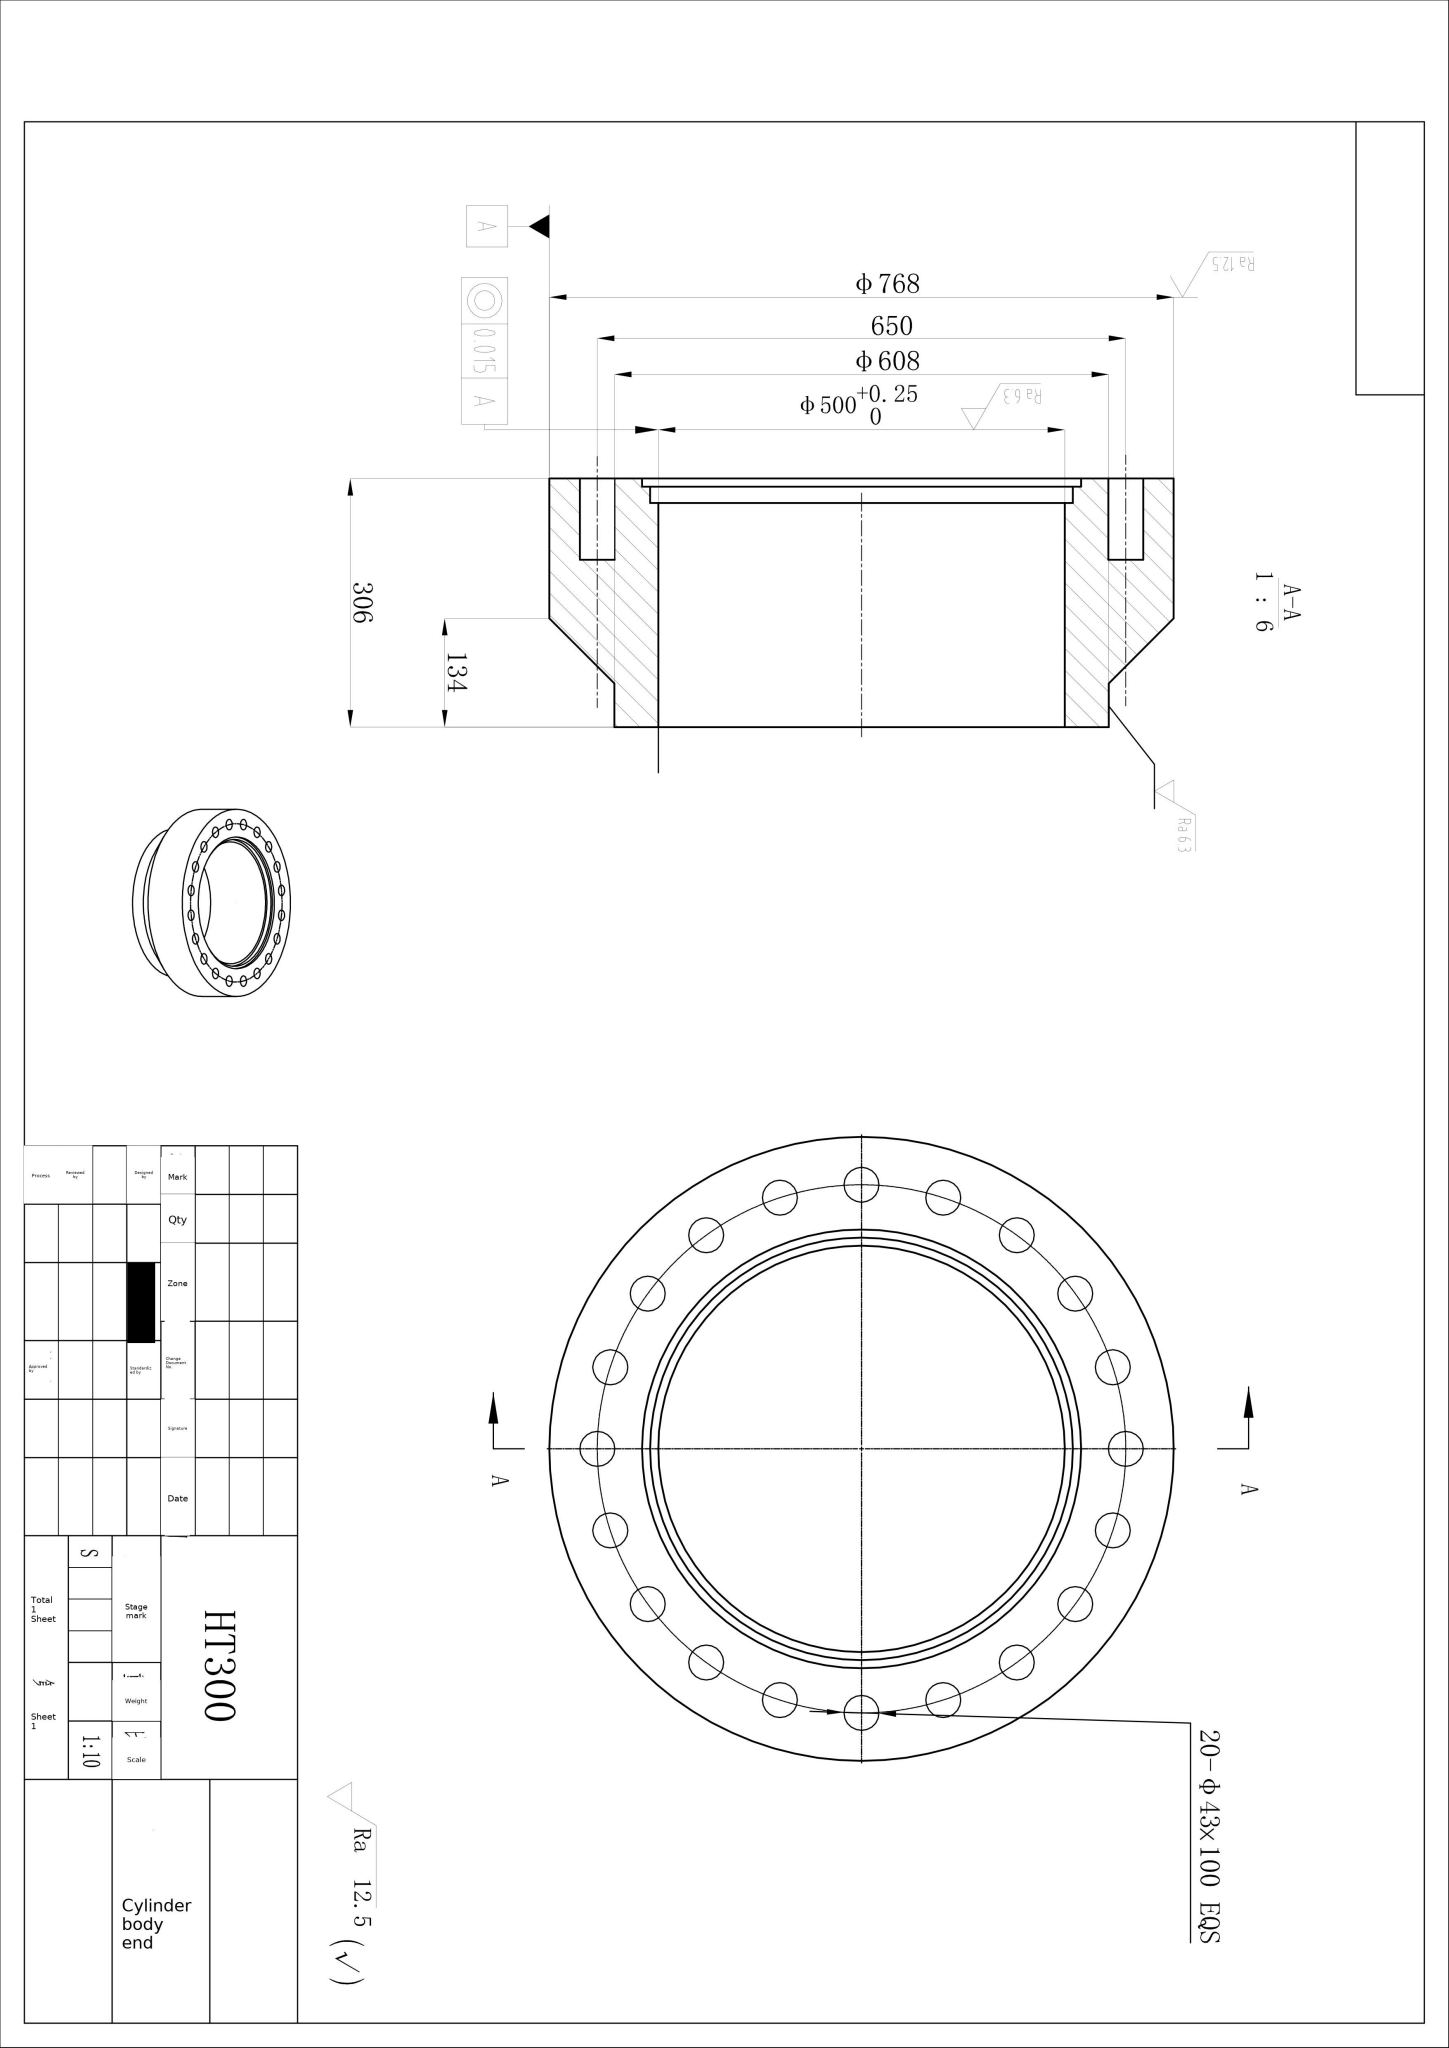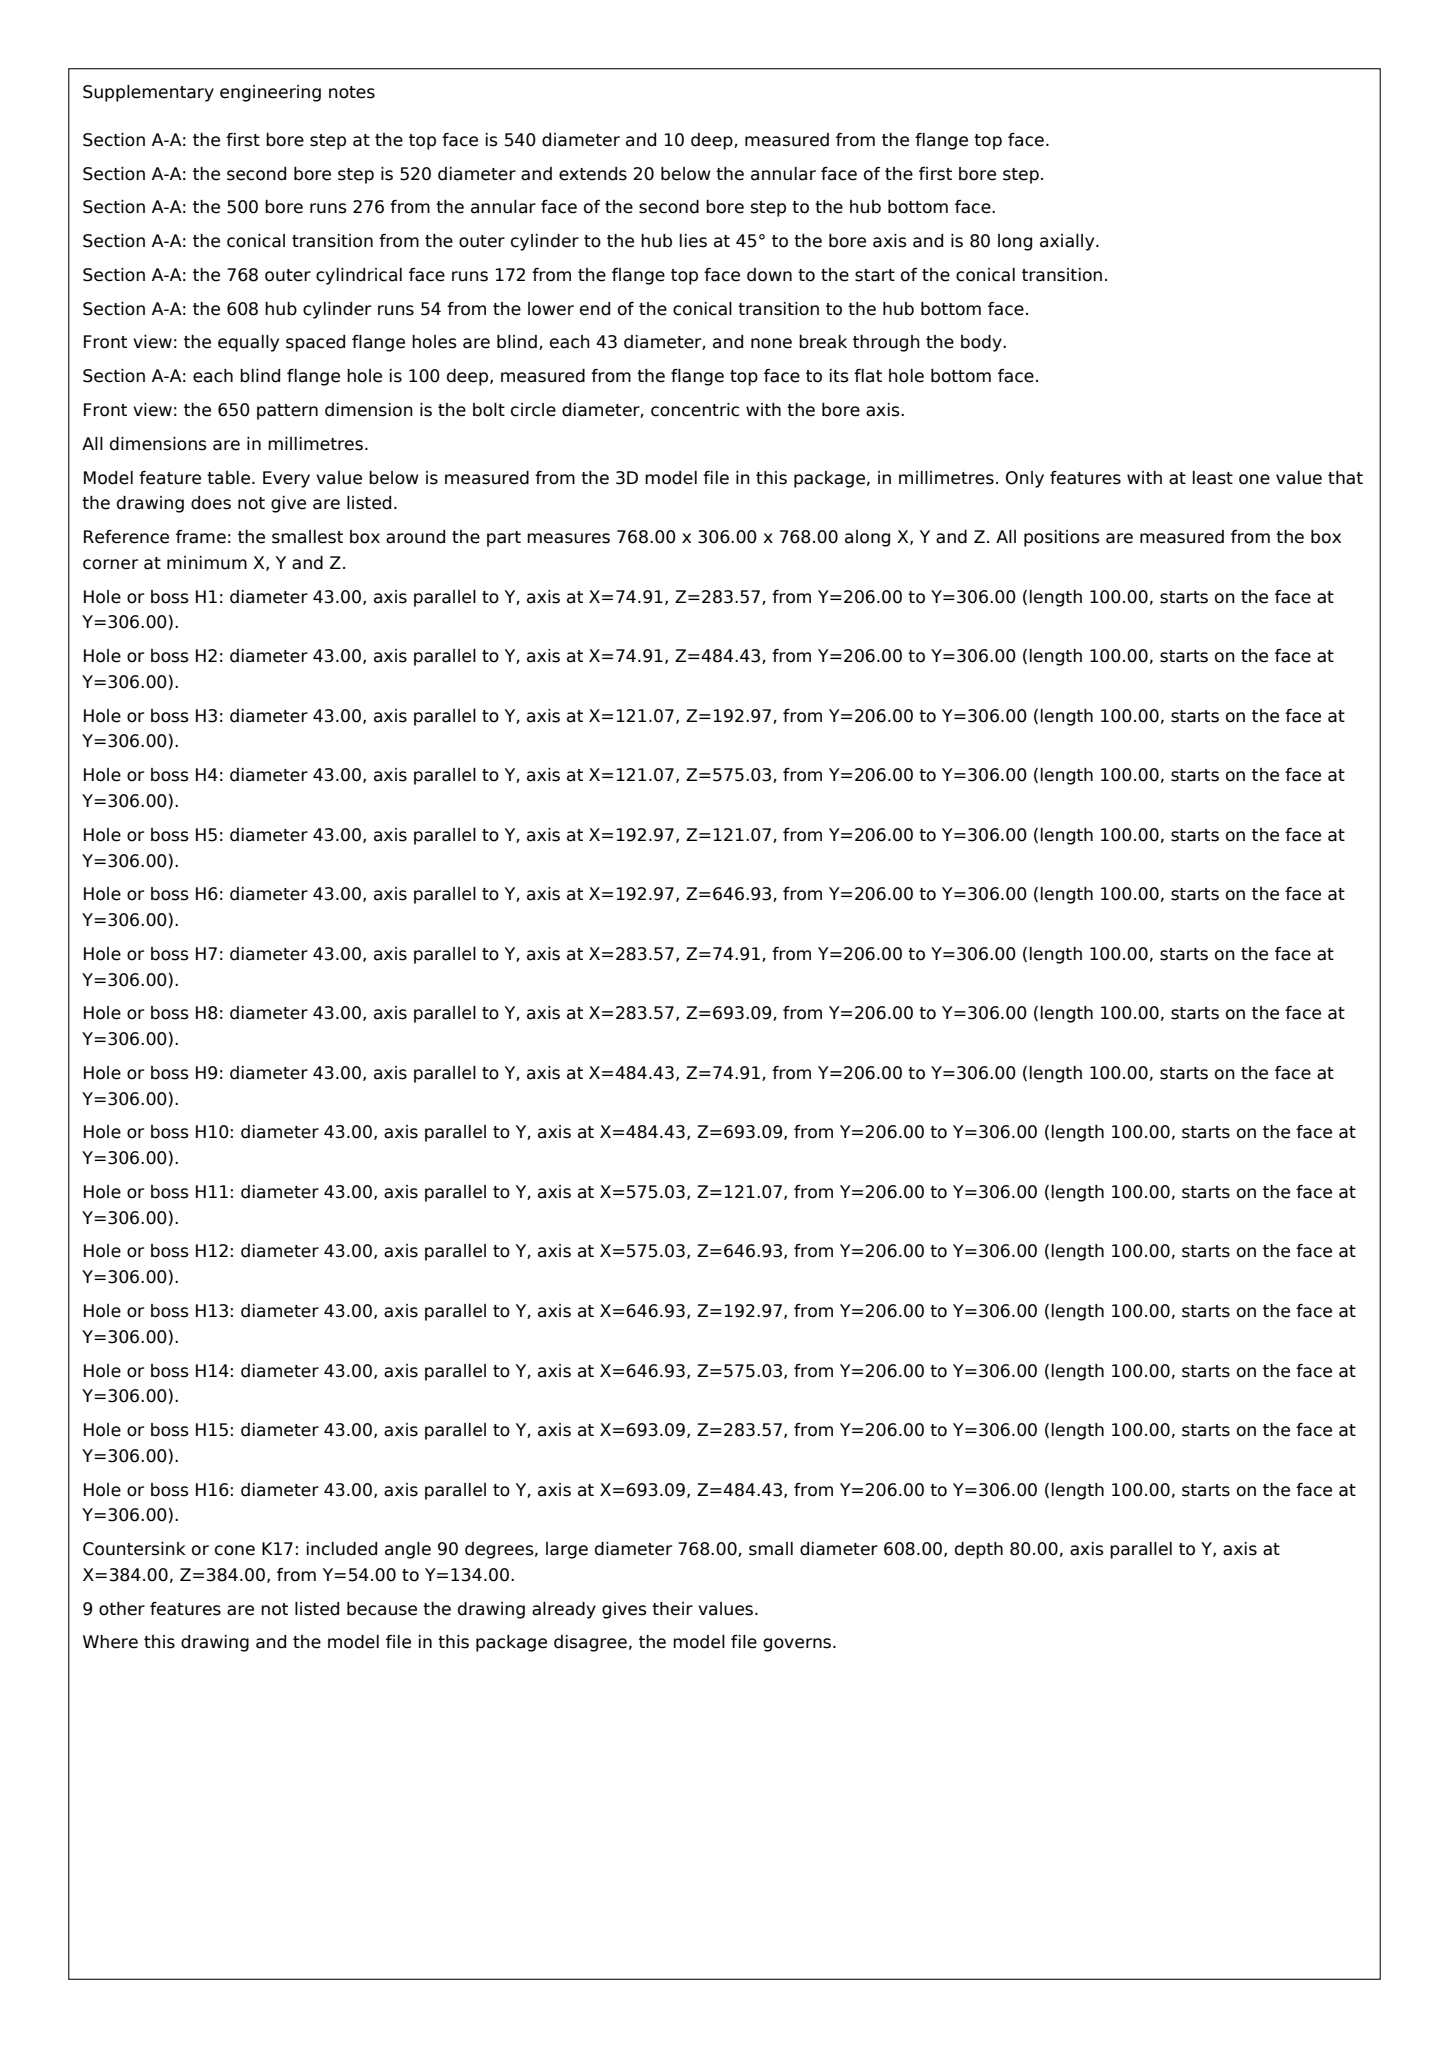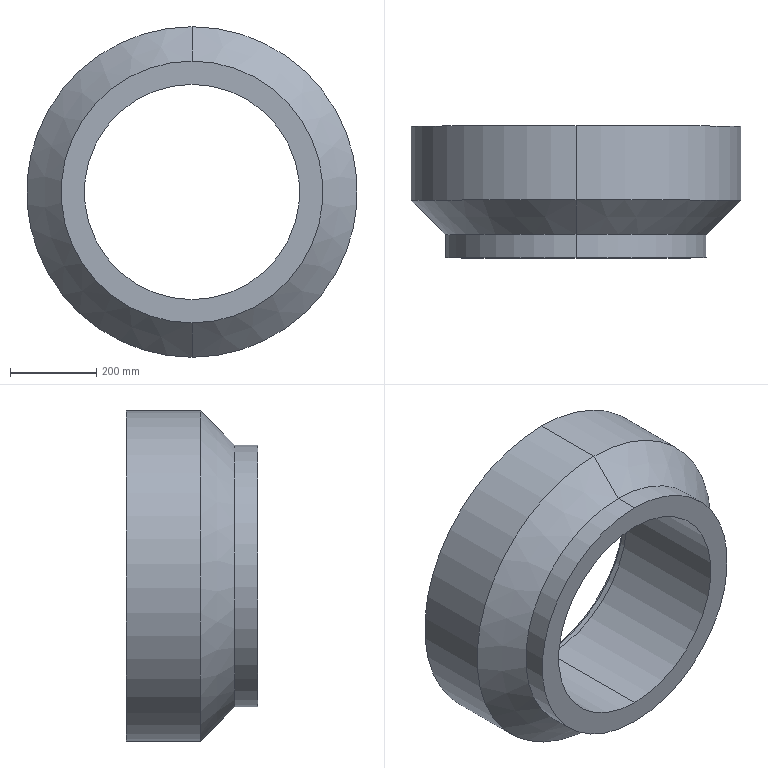Part | SolidWorks | mm | material HT300 | 1 solid | 76 faces | box 768 x 306 x 768 mm | volume 61597027 mm3 | cylinder 50 | plane 24 | cone 2 | commonest cylinder face diameters 43 x40 520 x2 500 x2 608 x2 768 x2 540 x2
Drawing notes:
CHAMFER Ø768 TO Ø608 AT LOWER END: 80 x 45° (C80) | from the solid: cones[90° incl, ref_dia 608]; Ø768 L172 + cone + Ø608 L54 = 306; (768-608)/2 = 80 leg
build123d program:
from build123d import *

# Parameters (mm, degrees)
SKETCH4_R          = 21.5
CUT_EXTRUDE1_DEPTH = 100


with BuildPart() as part:
    # Sketch1 → Revolve1 (revolve)
    with BuildSketch(Plane.XY, mode=Mode.PRIVATE) as revolve1_sk:
        Polygon((270, 0), (384, 0), (384, -172), (304, -252), (304, -306), (250, -306), (250, -30), (260, -30), (260, -10), (270, -10), align=None)
    revolve(revolve1_sk.sketch.rotate(Axis((0, 0, 0), (0, 1, 0)), 90), axis=Axis((0, 0, 0), (0, 1, 0)))

    # Sketch4 → Cut-Extrude1 (cut)
    with BuildSketch(Plane(origin=(0, 0, 0), x_dir=(1, 0, 0), z_dir=(0, 1, 0))):
        with Locations(Location((0, 325, 0), (0, 0, 270))):
            Circle(SKETCH4_R)
        with Locations(Location((100.431, 309.093, 0), (0, 0, 270))):
            Circle(SKETCH4_R)
        with Locations(Location((191.03, 262.931, 0), (0, 0, 270))):
            Circle(SKETCH4_R)
        with Locations(Location((262.931, 191.03, 0), (0, 0, 270))):
            Circle(SKETCH4_R)
        with Locations(Location((309.093, 100.431, 0), (0, 0, 270))):
            Circle(SKETCH4_R)
        with Locations(Location((325, 0, 0), (0, 0, 270))):
            Circle(SKETCH4_R)
        with Locations(Location((309.093, -100.431, 0), (0, 0, 270))):
            Circle(SKETCH4_R)
        with Locations(Location((262.931, -191.03, 0), (0, 0, 270))):
            Circle(SKETCH4_R)
        with Locations(Location((191.03, -262.931, 0), (0, 0, 270))):
            Circle(SKETCH4_R)
        with Locations(Location((100.431, -309.093, 0), (0, 0, 270))):
            Circle(SKETCH4_R)
        with Locations(Location((0, -325, 0), (0, 0, 270))):
            Circle(SKETCH4_R)
        with Locations(Location((-100.431, -309.093, 0), (0, 0, 270))):
            Circle(SKETCH4_R)
        with Locations(Location((-191.03, -262.931, 0), (0, 0, 270))):
            Circle(SKETCH4_R)
        with Locations(Location((-262.931, -191.03, 0), (0, 0, 270))):
            Circle(SKETCH4_R)
        with Locations(Location((-309.093, -100.431, 0), (0, 0, 270))):
            Circle(SKETCH4_R)
        with Locations(Location((-325, 0, 0), (0, 0, 270))):
            Circle(SKETCH4_R)
        with Locations(Location((-309.093, 100.431, 0), (0, 0, 270))):
            Circle(SKETCH4_R)
        with Locations(Location((-262.931, 191.03, 0), (0, 0, 270))):
            Circle(SKETCH4_R)
        with Locations(Location((-191.03, 262.931, 0), (0, 0, 270))):
            Circle(SKETCH4_R)
        with Locations(Location((-100.431, 309.093, 0), (0, 0, 270))):
            Circle(SKETCH4_R)
    extrude(amount=-CUT_EXTRUDE1_DEPTH, mode=Mode.SUBTRACT)


solid = part.part